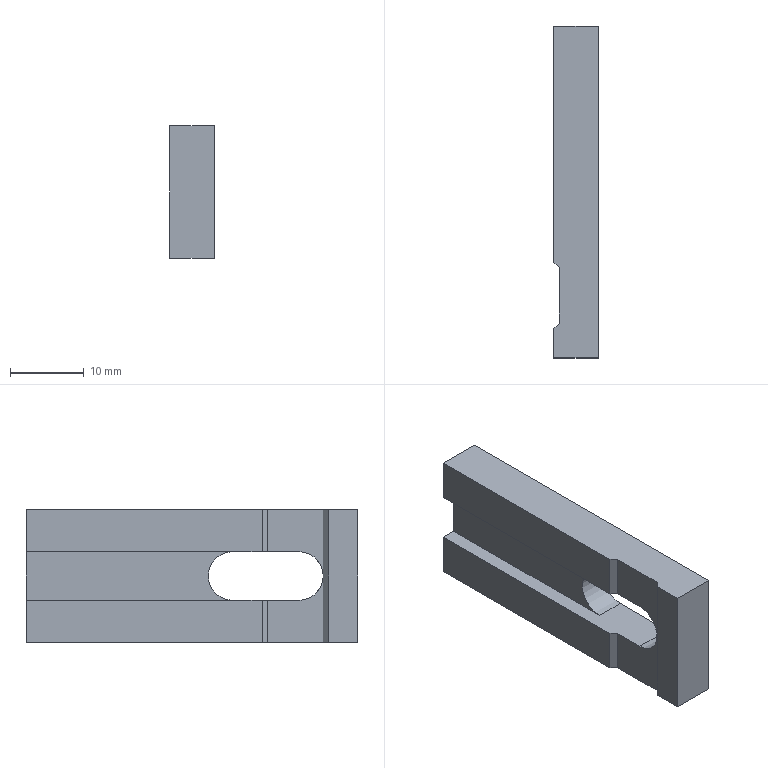Component | NX | CLAMP_PLATE_2 | 1 solid | 18 faces | volume 3887 mm3 | plane 16 | cylinder 2 | commonest cylinder face diameters 6.6 x2